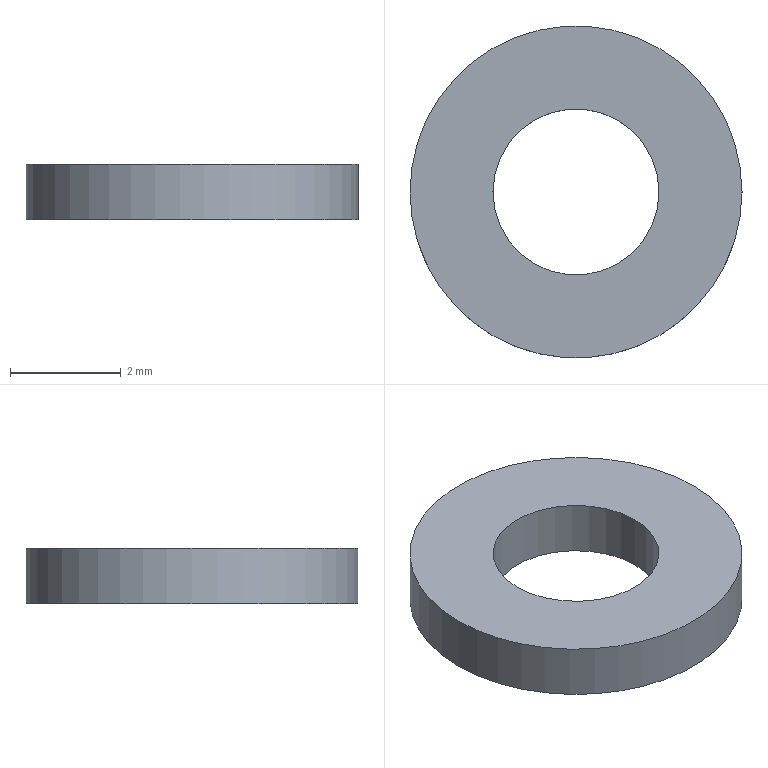Component | NX | EXT_PIPE_GASKET | 1 solid | 4 faces | volume 21 mm3 | cylinder 2 | plane 2 | commonest cylinder face diameters 6 x1 3 x1